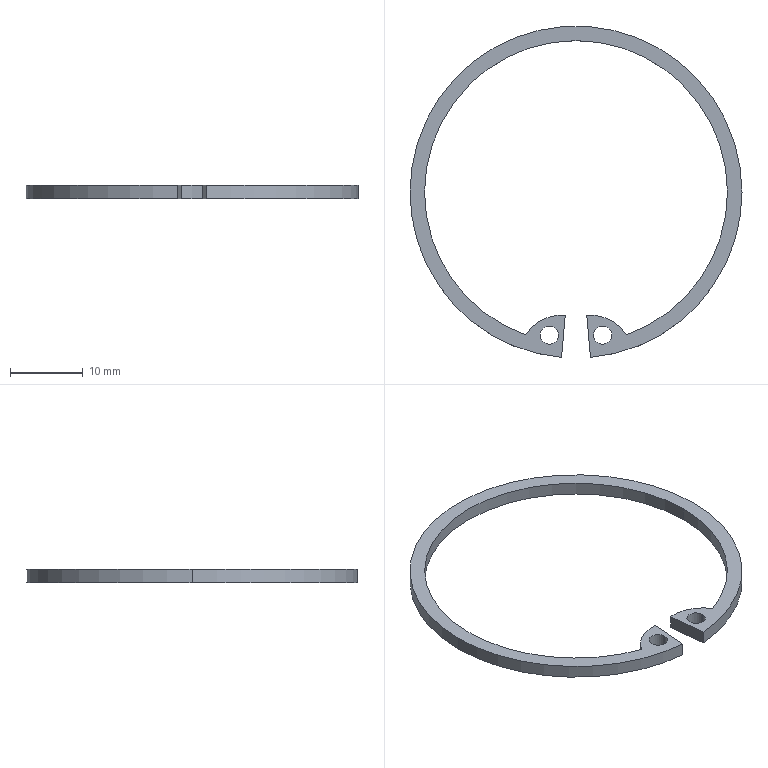Component | SolidWorks | BGRRB6905ZZ-1_RRING42-1 | 1 solid | 16 faces | box 45.5 x 45.41 x 1.8 mm | volume 510 mm3 | cylinder 12 | plane 4 | commonest cylinder face diameters 2.5 x4 41.5 x3 45.5 x3 11.6 x2 | material AISI 1045 Steel, cold drawn
build123d program:
from build123d import *

# Parameters (mm, degrees)
SKETCH1_R           = 1.25
BOSS_EXTRUDE1_DEPTH = 1.8


with BuildPart() as part:
    # Sketch1 → Boss-Extrude1 (new body)
    with BuildSketch(Plane.XY):
        with BuildLine():
            Line((-1.983, -22.663), (-1.477, -16.886))
            ThreePointArc((-1.477, -16.886), (-4.562, -17.468), (-6.891, -19.572))
            ThreePointArc((-6.891, -19.572), (0, 20.75), (6.891, -19.572))
            ThreePointArc((6.891, -19.572), (4.562, -17.468), (1.477, -16.886))
            Line((1.477, -16.886), (1.983, -22.663))
            ThreePointArc((1.983, -22.663), (0, 22.75), (-1.983, -22.663))
        make_face()
        with Locations((3.656, -19.606)):
            Circle(SKETCH1_R, mode=Mode.SUBTRACT)
        with Locations((-3.656, -19.606)):
            Circle(SKETCH1_R, mode=Mode.SUBTRACT)
    extrude(amount=BOSS_EXTRUDE1_DEPTH)


solid = part.part

# Placed as in the assembly
solid = solid.moved(Location((0, 0, 69), (0, 0, 0)))